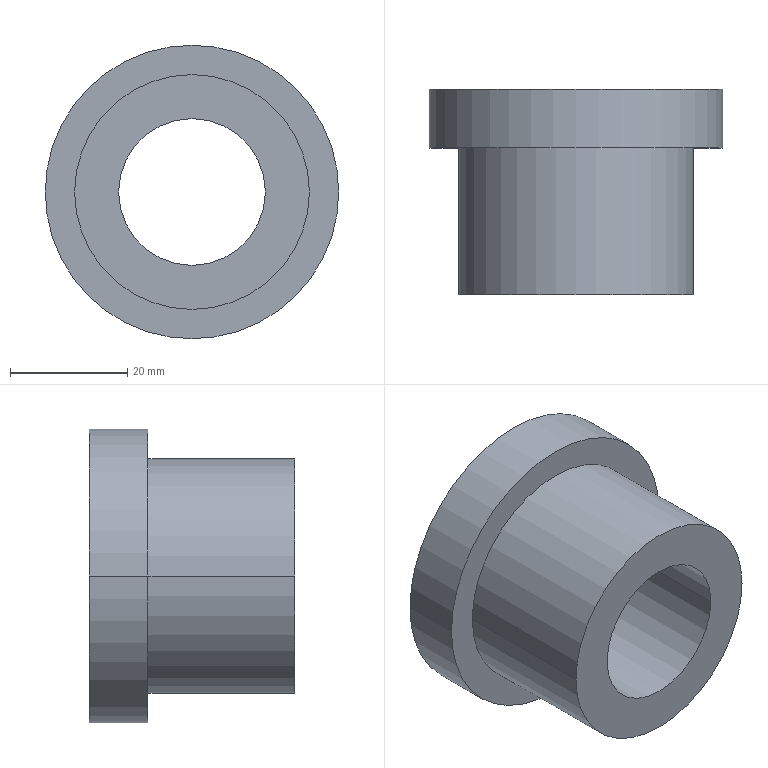Component | SolidWorks | LinearBearingSchematic-2 | 1 solid | 9 faces | box 50 x 35 x 50 mm | volume 33870 mm3 | cylinder 6 | plane 3 | commonest cylinder face diameters 50 x2 40 x2 25 x2
build123d program:
from build123d import *


with BuildPart() as part:
    # Sketch1 → Revolve1 (revolve)
    with BuildSketch(Plane(origin=(0, 0, 0), x_dir=(1, 0, 0), z_dir=(0, 1, 0)), mode=Mode.PRIVATE) as revolve1_sk:
        Polygon((-12.5, 0), (-20, 0), (-20, 25), (-25, 25), (-25, 35), (-12.5, 35), align=None)
    revolve(revolve1_sk.sketch.rotate(Axis((0, 0, 0), (0, 0, -1)), 180), axis=Axis((0, 0, 0), (0, 0, -1)))


solid = part.part

# Placed as in the assembly
solid = solid.moved(Location((-181.681, 803.438, 683.723), (90, 0, 0)))
STEP:
#1=COLOUR_RGB('',0.7922,0.8196,0.9333);
#2=FILL_AREA_STYLE_COLOUR('',#1);
#3=FILL_AREA_STYLE('',(#2));
#4=SURFACE_STYLE_FILL_AREA(#3);
#5=SURFACE_SIDE_STYLE('',(#4));
#6=SURFACE_STYLE_USAGE(.BOTH.,#5);
#7=PRESENTATION_STYLE_ASSIGNMENT((#6));
#8=CARTESIAN_POINT('',(-6.169,33.009,26.918));
#9=VERTEX_POINT('',#8);
#10=CARTESIAN_POINT('',(-8.137,33.009,26.918));
#11=VERTEX_POINT('',#10);
#12=CARTESIAN_POINT('',(-7.153,33.009,26.918));
#13=DIRECTION('',(0.,-1.,0.));
#14=DIRECTION('',(1.,0.,0.));
#15=AXIS2_PLACEMENT_3D('',#12,#13,#14);
#16=CIRCLE('',#15,0.9843);
#17=EDGE_CURVE('',#9,#11,#16,.T.);
#18=ORIENTED_EDGE('',*,*,#17,.T.);
#19=CARTESIAN_POINT('',(-8.137,32.616,26.918));
#20=VERTEX_POINT('',#19);
#21=CARTESIAN_POINT('',(-8.137,31.631,26.918));
#22=DIRECTION('',(0.,-1.,0.));
#23=VECTOR('',#22,39.37);
#24=LINE('',#21,#23);
#25=EDGE_CURVE('',#11,#20,#24,.T.);
#26=ORIENTED_EDGE('',*,*,#25,.T.);
#27=CARTESIAN_POINT('',(-6.169,32.616,26.918));
#28=VERTEX_POINT('',#27);
#29=CARTESIAN_POINT('',(-7.153,32.616,26.918));
#30=DIRECTION('',(0.,-1.,0.));
#31=DIRECTION('',(1.,0.,0.));
#32=AXIS2_PLACEMENT_3D('',#29,#30,#31);
#33=CIRCLE('',#32,0.9843);
#34=EDGE_CURVE('',#28,#20,#33,.T.);
#35=ORIENTED_EDGE('',*,*,#34,.F.);
#36=CARTESIAN_POINT('',(-6.169,31.631,26.918));
#37=DIRECTION('',(0.,-1.,0.));
#38=VECTOR('',#37,39.37);
#39=LINE('',#36,#38);
#40=EDGE_CURVE('',#9,#28,#39,.T.);
#41=ORIENTED_EDGE('',*,*,#40,.F.);
#42=EDGE_LOOP('',(#18,#26,#35,#41));
#43=FACE_OUTER_BOUND('',#42,.T.);
#44=CARTESIAN_POINT('',(-7.153,31.631,26.918));
#45=DIRECTION('',(0.,-1.,0.));
#46=DIRECTION('',(1.,0.,0.));
#47=AXIS2_PLACEMENT_3D('',#44,#45,#46);
#48=CYLINDRICAL_SURFACE('',#47,0.9843);
#49=ADVANCED_FACE('',(#43),#48,.T.);
#50=CARTESIAN_POINT('',(-6.365,32.616,26.918));
#51=VERTEX_POINT('',#50);
#52=CARTESIAN_POINT('',(-7.94,32.616,26.918));
#53=VERTEX_POINT('',#52);
#54=CARTESIAN_POINT('',(-7.153,32.616,26.918));
#55=DIRECTION('',(0.,-1.,0.));
#56=DIRECTION('',(1.,0.,0.));
#57=AXIS2_PLACEMENT_3D('',#54,#55,#56);
#58=CIRCLE('',#57,0.7874);
#59=EDGE_CURVE('',#51,#53,#58,.T.);
#60=ORIENTED_EDGE('',*,*,#59,.T.);
#61=CARTESIAN_POINT('',(-7.94,31.631,26.918));
#62=VERTEX_POINT('',#61);
#63=CARTESIAN_POINT('',(-7.94,31.631,26.918));
#64=DIRECTION('',(0.,-1.,0.));
#65=VECTOR('',#64,39.37);
#66=LINE('',#63,#65);
#67=EDGE_CURVE('',#53,#62,#66,.T.);
#68=ORIENTED_EDGE('',*,*,#67,.T.);
#69=CARTESIAN_POINT('',(-6.365,31.631,26.918));
#70=VERTEX_POINT('',#69);
#71=CARTESIAN_POINT('',(-7.153,31.631,26.918));
#72=DIRECTION('',(0.,-1.,0.));
#73=DIRECTION('',(1.,0.,0.));
#74=AXIS2_PLACEMENT_3D('',#71,#72,#73);
#75=CIRCLE('',#74,0.7874);
#76=EDGE_CURVE('',#70,#62,#75,.T.);
#77=ORIENTED_EDGE('',*,*,#76,.F.);
#78=CARTESIAN_POINT('',(-6.365,31.631,26.918));
#79=DIRECTION('',(0.,-1.,0.));
#80=VECTOR('',#79,39.37);
#81=LINE('',#78,#80);
#82=EDGE_CURVE('',#51,#70,#81,.T.);
#83=ORIENTED_EDGE('',*,*,#82,.F.);
#84=EDGE_LOOP('',(#60,#68,#77,#83));
#85=FACE_OUTER_BOUND('',#84,.T.);
#86=CARTESIAN_POINT('',(-7.153,31.631,26.918));
#87=DIRECTION('',(0.,-1.,0.));
#88=DIRECTION('',(1.,0.,0.));
#89=AXIS2_PLACEMENT_3D('',#86,#87,#88);
#90=CYLINDRICAL_SURFACE('',#89,0.7874);
#91=ADVANCED_FACE('',(#85),#90,.T.);
#92=CARTESIAN_POINT('',(-7.645,33.009,26.918));
#93=VERTEX_POINT('',#92);
#94=CARTESIAN_POINT('',(-6.661,33.009,26.918));
#95=VERTEX_POINT('',#94);
#96=CARTESIAN_POINT('',(-7.153,33.009,26.918));
#97=DIRECTION('',(0.,-1.,0.));
#98=DIRECTION('',(1.,0.,0.));
#99=AXIS2_PLACEMENT_3D('',#96,#97,#98);
#100=CIRCLE('',#99,0.4921);
#101=EDGE_CURVE('',#93,#95,#100,.T.);
#102=ORIENTED_EDGE('',*,*,#101,.F.);
#103=CARTESIAN_POINT('',(-7.645,31.631,26.918));
#104=VERTEX_POINT('',#103);
#105=CARTESIAN_POINT('',(-7.645,31.631,26.918));
#106=DIRECTION('',(0.,-1.,0.));
#107=VECTOR('',#106,39.37);
#108=LINE('',#105,#107);
#109=EDGE_CURVE('',#93,#104,#108,.T.);
#110=ORIENTED_EDGE('',*,*,#109,.T.);
#111=CARTESIAN_POINT('',(-6.661,31.631,26.918));
#112=VERTEX_POINT('',#111);
#113=CARTESIAN_POINT('',(-7.153,31.631,26.918));
#114=DIRECTION('',(0.,-1.,0.));
#115=DIRECTION('',(1.,0.,0.));
#116=AXIS2_PLACEMENT_3D('',#113,#114,#115);
#117=CIRCLE('',#116,0.4921);
#118=EDGE_CURVE('',#104,#112,#117,.T.);
#119=ORIENTED_EDGE('',*,*,#118,.T.);
#120=CARTESIAN_POINT('',(-6.661,31.631,26.918));
#121=DIRECTION('',(0.,-1.,0.));
#122=VECTOR('',#121,39.37);
#123=LINE('',#120,#122);
#124=EDGE_CURVE('',#95,#112,#123,.T.);
#125=ORIENTED_EDGE('',*,*,#124,.F.);
#126=EDGE_LOOP('',(#102,#110,#119,#125));
#127=FACE_OUTER_BOUND('',#126,.T.);
#128=CARTESIAN_POINT('',(-7.153,31.631,26.918));
#129=DIRECTION('',(0.,-1.,0.));
#130=DIRECTION('',(1.,0.,0.));
#131=AXIS2_PLACEMENT_3D('',#128,#129,#130);
#132=CYLINDRICAL_SURFACE('',#131,0.4921);
#133=ADVANCED_FACE('',(#127),#132,.F.);
#134=ORIENTED_EDGE('',*,*,#109,.F.);
#135=CARTESIAN_POINT('',(-7.153,33.009,26.918));
#136=DIRECTION('',(0.,-1.,0.));
#137=DIRECTION('',(1.,0.,0.));
#138=AXIS2_PLACEMENT_3D('',#135,#136,#137);
#139=CIRCLE('',#138,0.4921);
#140=EDGE_CURVE('',#95,#93,#139,.T.);
#141=ORIENTED_EDGE('',*,*,#140,.F.);
#142=ORIENTED_EDGE('',*,*,#124,.T.);
#143=CARTESIAN_POINT('',(-7.153,31.631,26.918));
#144=DIRECTION('',(0.,-1.,0.));
#145=DIRECTION('',(1.,0.,0.));
#146=AXIS2_PLACEMENT_3D('',#143,#144,#145);
#147=CIRCLE('',#146,0.4921);
#148=EDGE_CURVE('',#112,#104,#147,.T.);
#149=ORIENTED_EDGE('',*,*,#148,.T.);
#150=EDGE_LOOP('',(#134,#141,#142,#149));
#151=FACE_OUTER_BOUND('',#150,.T.);
#152=CARTESIAN_POINT('',(-7.153,31.631,26.918));
#153=DIRECTION('',(0.,-1.,0.));
#154=DIRECTION('',(1.,0.,0.));
#155=AXIS2_PLACEMENT_3D('',#152,#153,#154);
#156=CYLINDRICAL_SURFACE('',#155,0.4921);
#157=ADVANCED_FACE('',(#151),#156,.F.);
#158=ORIENTED_EDGE('',*,*,#148,.F.);
#159=ORIENTED_EDGE('',*,*,#118,.F.);
#160=EDGE_LOOP('',(#158,#159));
#161=FACE_BOUND('',#160,.T.);
#162=ORIENTED_EDGE('',*,*,#76,.T.);
#163=CARTESIAN_POINT('',(-7.153,31.631,26.918));
#164=DIRECTION('',(0.,-1.,0.));
#165=DIRECTION('',(1.,0.,0.));
#166=AXIS2_PLACEMENT_3D('',#163,#164,#165);
#167=CIRCLE('',#166,0.7874);
#168=EDGE_CURVE('',#62,#70,#167,.T.);
#169=ORIENTED_EDGE('',*,*,#168,.T.);
#170=EDGE_LOOP('',(#162,#169));
#171=FACE_OUTER_BOUND('',#170,.T.);
#172=CARTESIAN_POINT('',(-7.645,31.631,26.918));
#173=DIRECTION('',(0.,1.,0.));
#174=DIRECTION('',(-1.,0.,0.));
#175=AXIS2_PLACEMENT_3D('',#172,#173,#174);
#176=PLANE('',#175);
#177=ADVANCED_FACE('',(#161,#171),#176,.F.);
#178=ORIENTED_EDGE('',*,*,#67,.F.);
#179=CARTESIAN_POINT('',(-7.153,32.616,26.918));
#180=DIRECTION('',(0.,-1.,0.));
#181=DIRECTION('',(1.,0.,0.));
#182=AXIS2_PLACEMENT_3D('',#179,#180,#181);
#183=CIRCLE('',#182,0.7874);
#184=EDGE_CURVE('',#53,#51,#183,.T.);
#185=ORIENTED_EDGE('',*,*,#184,.T.);
#186=ORIENTED_EDGE('',*,*,#82,.T.);
#187=ORIENTED_EDGE('',*,*,#168,.F.);
#188=EDGE_LOOP('',(#178,#185,#186,#187));
#189=FACE_OUTER_BOUND('',#188,.T.);
#190=CARTESIAN_POINT('',(-7.153,31.631,26.918));
#191=DIRECTION('',(0.,-1.,0.));
#192=DIRECTION('',(1.,0.,0.));
#193=AXIS2_PLACEMENT_3D('',#190,#191,#192);
#194=CYLINDRICAL_SURFACE('',#193,0.7874);
#195=ADVANCED_FACE('',(#189),#194,.T.);
#196=ORIENTED_EDGE('',*,*,#59,.F.);
#197=ORIENTED_EDGE('',*,*,#184,.F.);
#198=EDGE_LOOP('',(#196,#197));
#199=FACE_BOUND('',#198,.T.);
#200=ORIENTED_EDGE('',*,*,#34,.T.);
#201=CARTESIAN_POINT('',(-7.153,32.616,26.918));
#202=DIRECTION('',(0.,-1.,0.));
#203=DIRECTION('',(1.,0.,0.));
#204=AXIS2_PLACEMENT_3D('',#201,#202,#203);
#205=CIRCLE('',#204,0.9843);
#206=EDGE_CURVE('',#20,#28,#205,.T.);
#207=ORIENTED_EDGE('',*,*,#206,.T.);
#208=EDGE_LOOP('',(#200,#207));
#209=FACE_OUTER_BOUND('',#208,.T.);
#210=CARTESIAN_POINT('',(-7.94,32.616,26.918));
#211=DIRECTION('',(0.,1.,0.));
#212=DIRECTION('',(-1.,0.,0.));
#213=AXIS2_PLACEMENT_3D('',#210,#211,#212);
#214=PLANE('',#213);
#215=ADVANCED_FACE('',(#199,#209),#214,.F.);
#216=ORIENTED_EDGE('',*,*,#25,.F.);
#217=CARTESIAN_POINT('',(-7.153,33.009,26.918));
#218=DIRECTION('',(0.,-1.,0.));
#219=DIRECTION('',(1.,0.,0.));
#220=AXIS2_PLACEMENT_3D('',#217,#218,#219);
#221=CIRCLE('',#220,0.9843);
#222=EDGE_CURVE('',#11,#9,#221,.T.);
#223=ORIENTED_EDGE('',*,*,#222,.T.);
#224=ORIENTED_EDGE('',*,*,#40,.T.);
#225=ORIENTED_EDGE('',*,*,#206,.F.);
#226=EDGE_LOOP('',(#216,#223,#224,#225));
#227=FACE_OUTER_BOUND('',#226,.T.);
#228=CARTESIAN_POINT('',(-7.153,31.631,26.918));
#229=DIRECTION('',(0.,-1.,0.));
#230=DIRECTION('',(1.,0.,0.));
#231=AXIS2_PLACEMENT_3D('',#228,#229,#230);
#232=CYLINDRICAL_SURFACE('',#231,0.9843);
#233=ADVANCED_FACE('',(#227),#232,.T.);
#234=ORIENTED_EDGE('',*,*,#17,.F.);
#235=ORIENTED_EDGE('',*,*,#222,.F.);
#236=EDGE_LOOP('',(#234,#235));
#237=FACE_OUTER_BOUND('',#236,.T.);
#238=ORIENTED_EDGE('',*,*,#140,.T.);
#239=ORIENTED_EDGE('',*,*,#101,.T.);
#240=EDGE_LOOP('',(#238,#239));
#241=FACE_BOUND('',#240,.T.);
#242=CARTESIAN_POINT('',(-8.137,33.009,26.918));
#243=DIRECTION('',(0.,-1.,0.));
#244=DIRECTION('',(1.,0.,0.));
#245=AXIS2_PLACEMENT_3D('',#242,#243,#244);
#246=PLANE('',#245);
#247=ADVANCED_FACE('',(#237,#241),#246,.F.);
#248=CLOSED_SHELL('',(#49,#91,#133,#157,#177,#195,#215,#233,#247));
#249=MANIFOLD_SOLID_BREP('',#248);
#250=STYLED_ITEM('',(#7),#249);
#251=PRESENTATION_LAYER_ASSIGNMENT('','',(#250));
#252=CARTESIAN_POINT('',(0.,0.,0.));
#253=DIRECTION('',(0.,0.,1.));
#254=DIRECTION('',(1.,0.,0.));
#255=AXIS2_PLACEMENT_3D('',#252,#253,#254);
#256=(LENGTH_UNIT()NAMED_UNIT(*)SI_UNIT($,.METRE.));
#257=LENGTH_MEASURE_WITH_UNIT(LENGTH_MEASURE(0.0254),#256);
#258=DIMENSIONAL_EXPONENTS(1.,0.,0.,0.,0.,0.,0.);
#259=(CONVERSION_BASED_UNIT('',#257)LENGTH_UNIT()NAMED_UNIT(#258));
#260=UNCERTAINTY_MEASURE_WITH_UNIT(LENGTH_MEASURE(0.00001),#259,'','');
#261=(NAMED_UNIT(*)PLANE_ANGLE_UNIT()SI_UNIT($,.RADIAN.));
#262=(NAMED_UNIT(*)SI_UNIT($,.STERADIAN.)SOLID_ANGLE_UNIT());
#263=(GEOMETRIC_REPRESENTATION_CONTEXT(3)GLOBAL_UNCERTAINTY_ASSIGNED_CONTEXT((#260))GLOBAL_UNIT_ASSIGNED_CONTEXT((#259,#261,#262))REPRESENTATION_CONTEXT('',''));
#264=ADVANCED_BREP_SHAPE_REPRESENTATION('',(#249,#255),#263);
#265=(LENGTH_UNIT()NAMED_UNIT(*)SI_UNIT($,.METRE.));
#266=LENGTH_MEASURE_WITH_UNIT(LENGTH_MEASURE(0.0254),#265);
#267=DIMENSIONAL_EXPONENTS(1.,0.,0.,0.,0.,0.,0.);
#268=(CONVERSION_BASED_UNIT('',#266)LENGTH_UNIT()NAMED_UNIT(#267));
#269=UNCERTAINTY_MEASURE_WITH_UNIT(LENGTH_MEASURE(0.00001),#268,'','');
#270=(NAMED_UNIT(*)PLANE_ANGLE_UNIT()SI_UNIT($,.RADIAN.));
#271=(NAMED_UNIT(*)SI_UNIT($,.STERADIAN.)SOLID_ANGLE_UNIT());
#272=(GEOMETRIC_REPRESENTATION_CONTEXT(3)GLOBAL_UNCERTAINTY_ASSIGNED_CONTEXT((#269))GLOBAL_UNIT_ASSIGNED_CONTEXT((#268,#270,#271))REPRESENTATION_CONTEXT('',''));
#273=MECHANICAL_DESIGN_GEOMETRIC_PRESENTATION_REPRESENTATION('',(#250),#272);